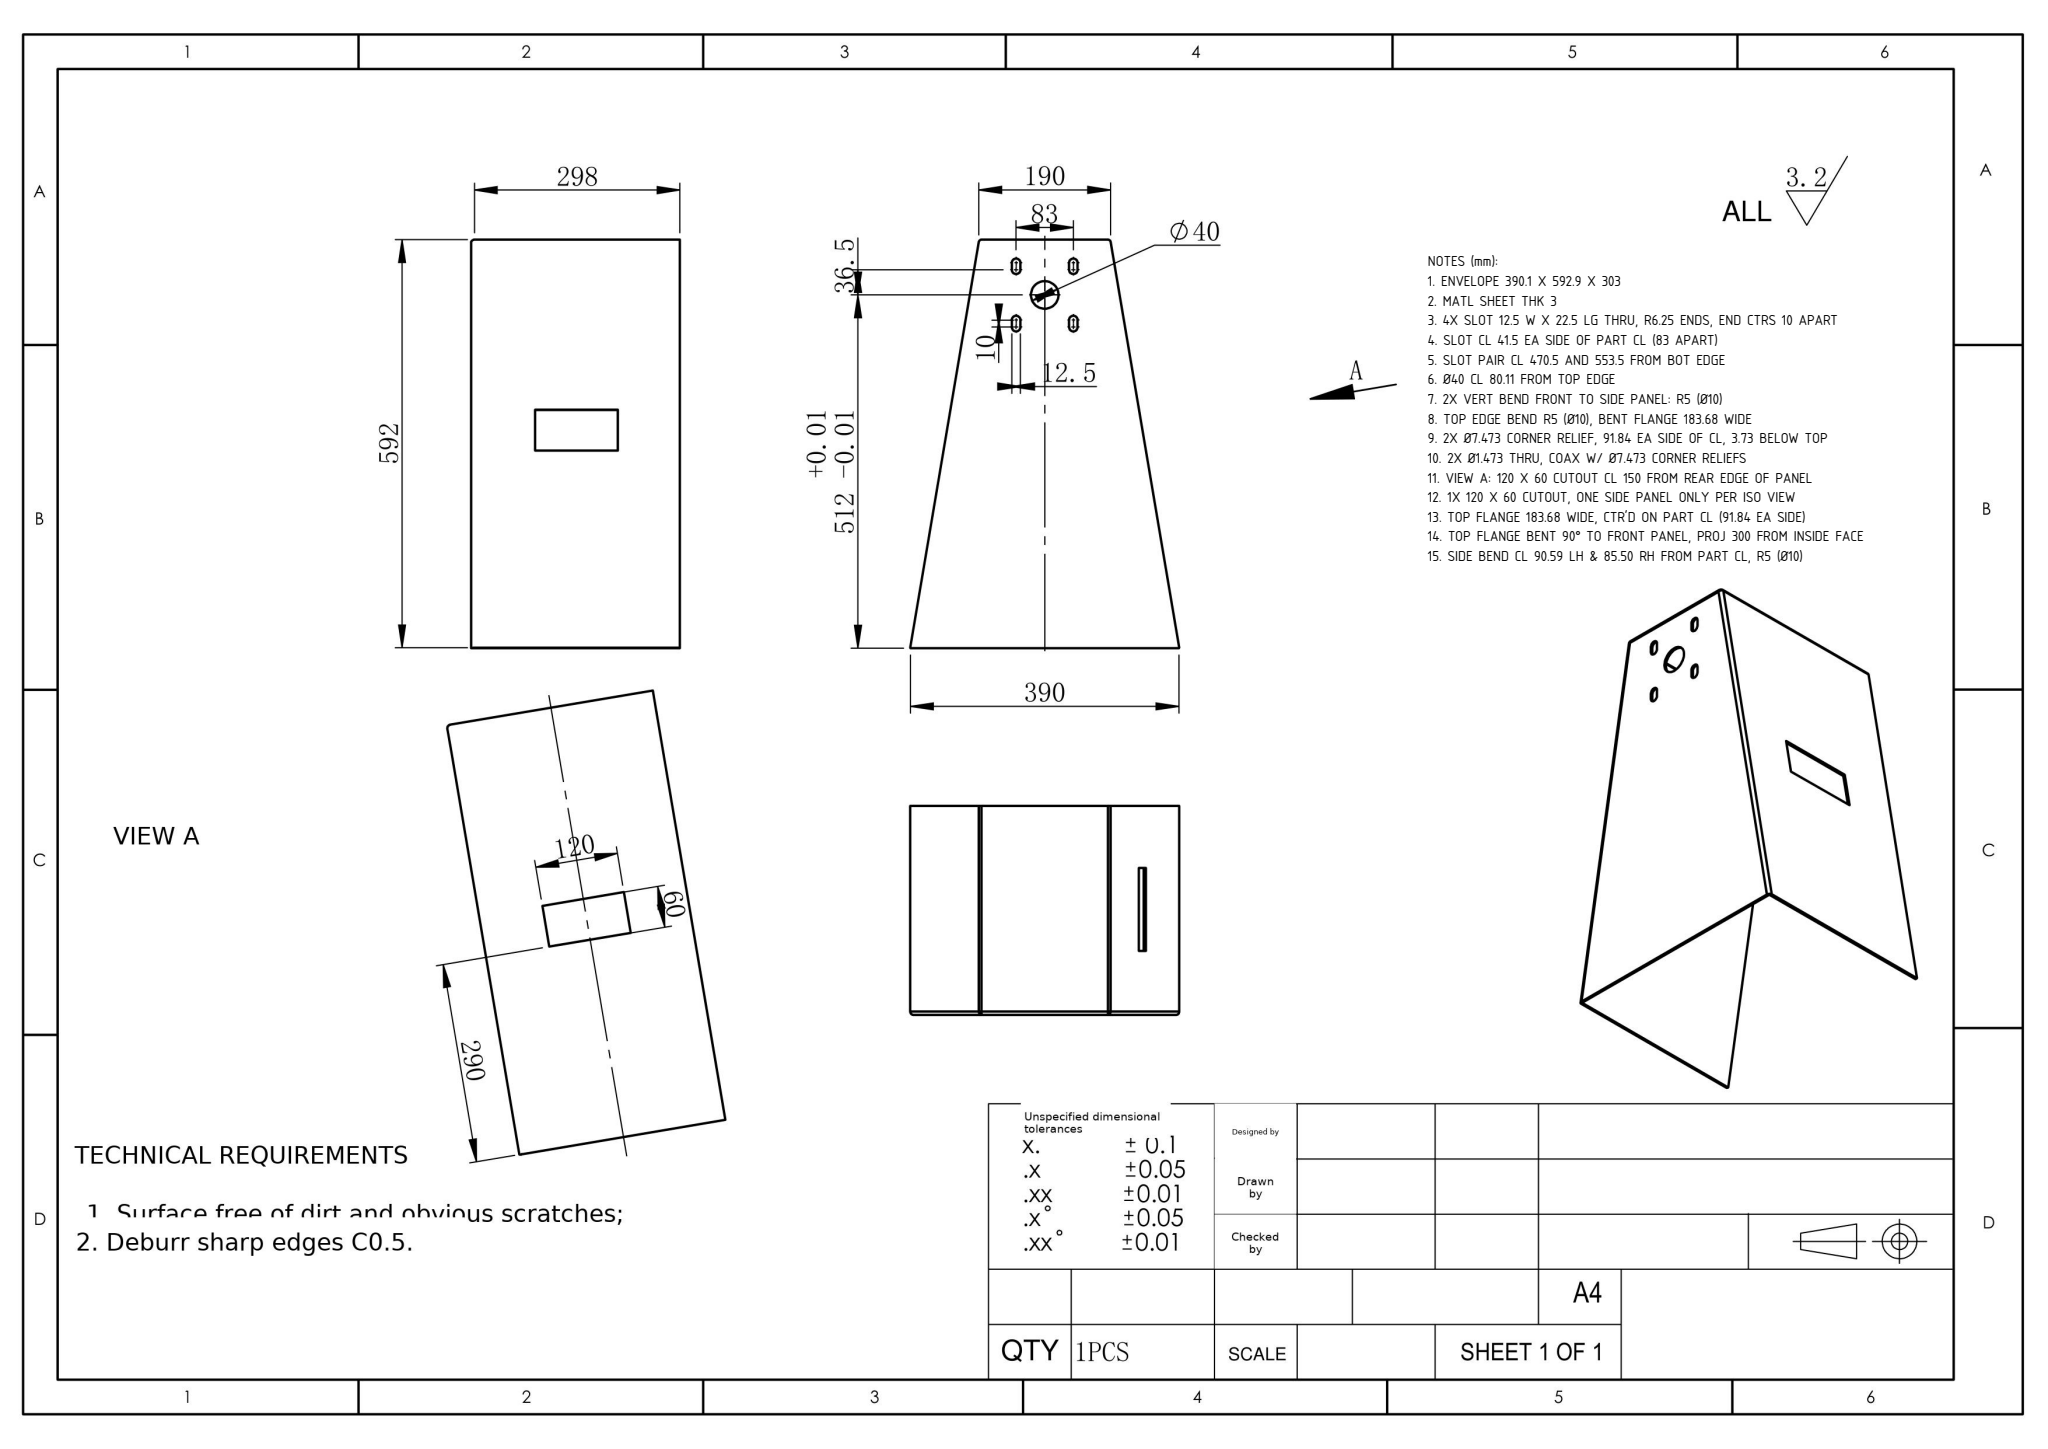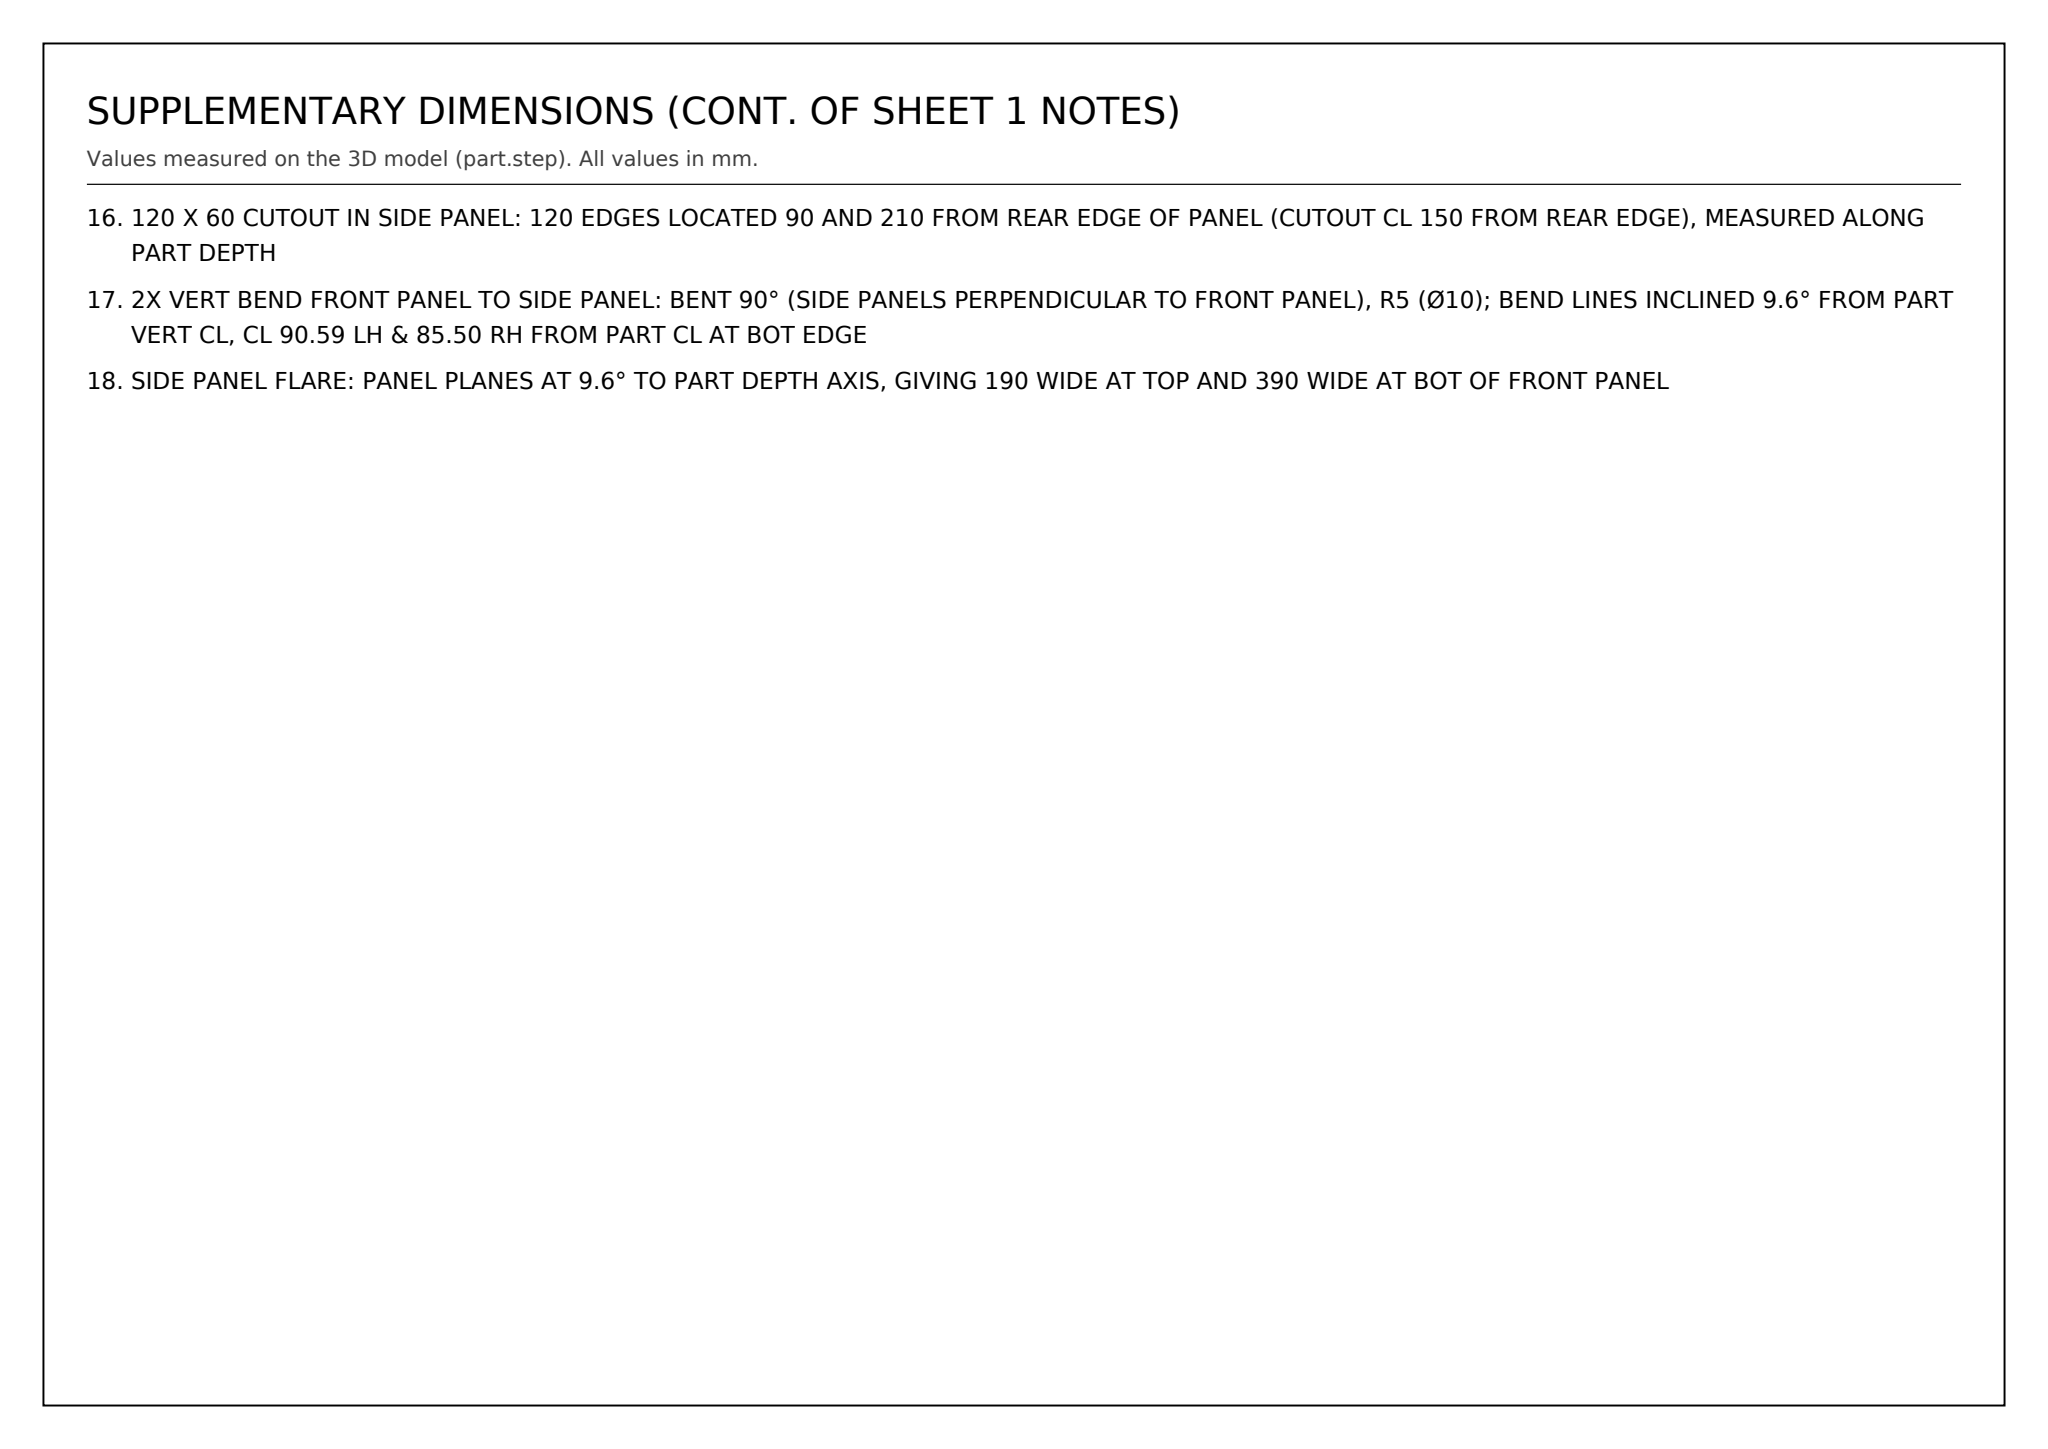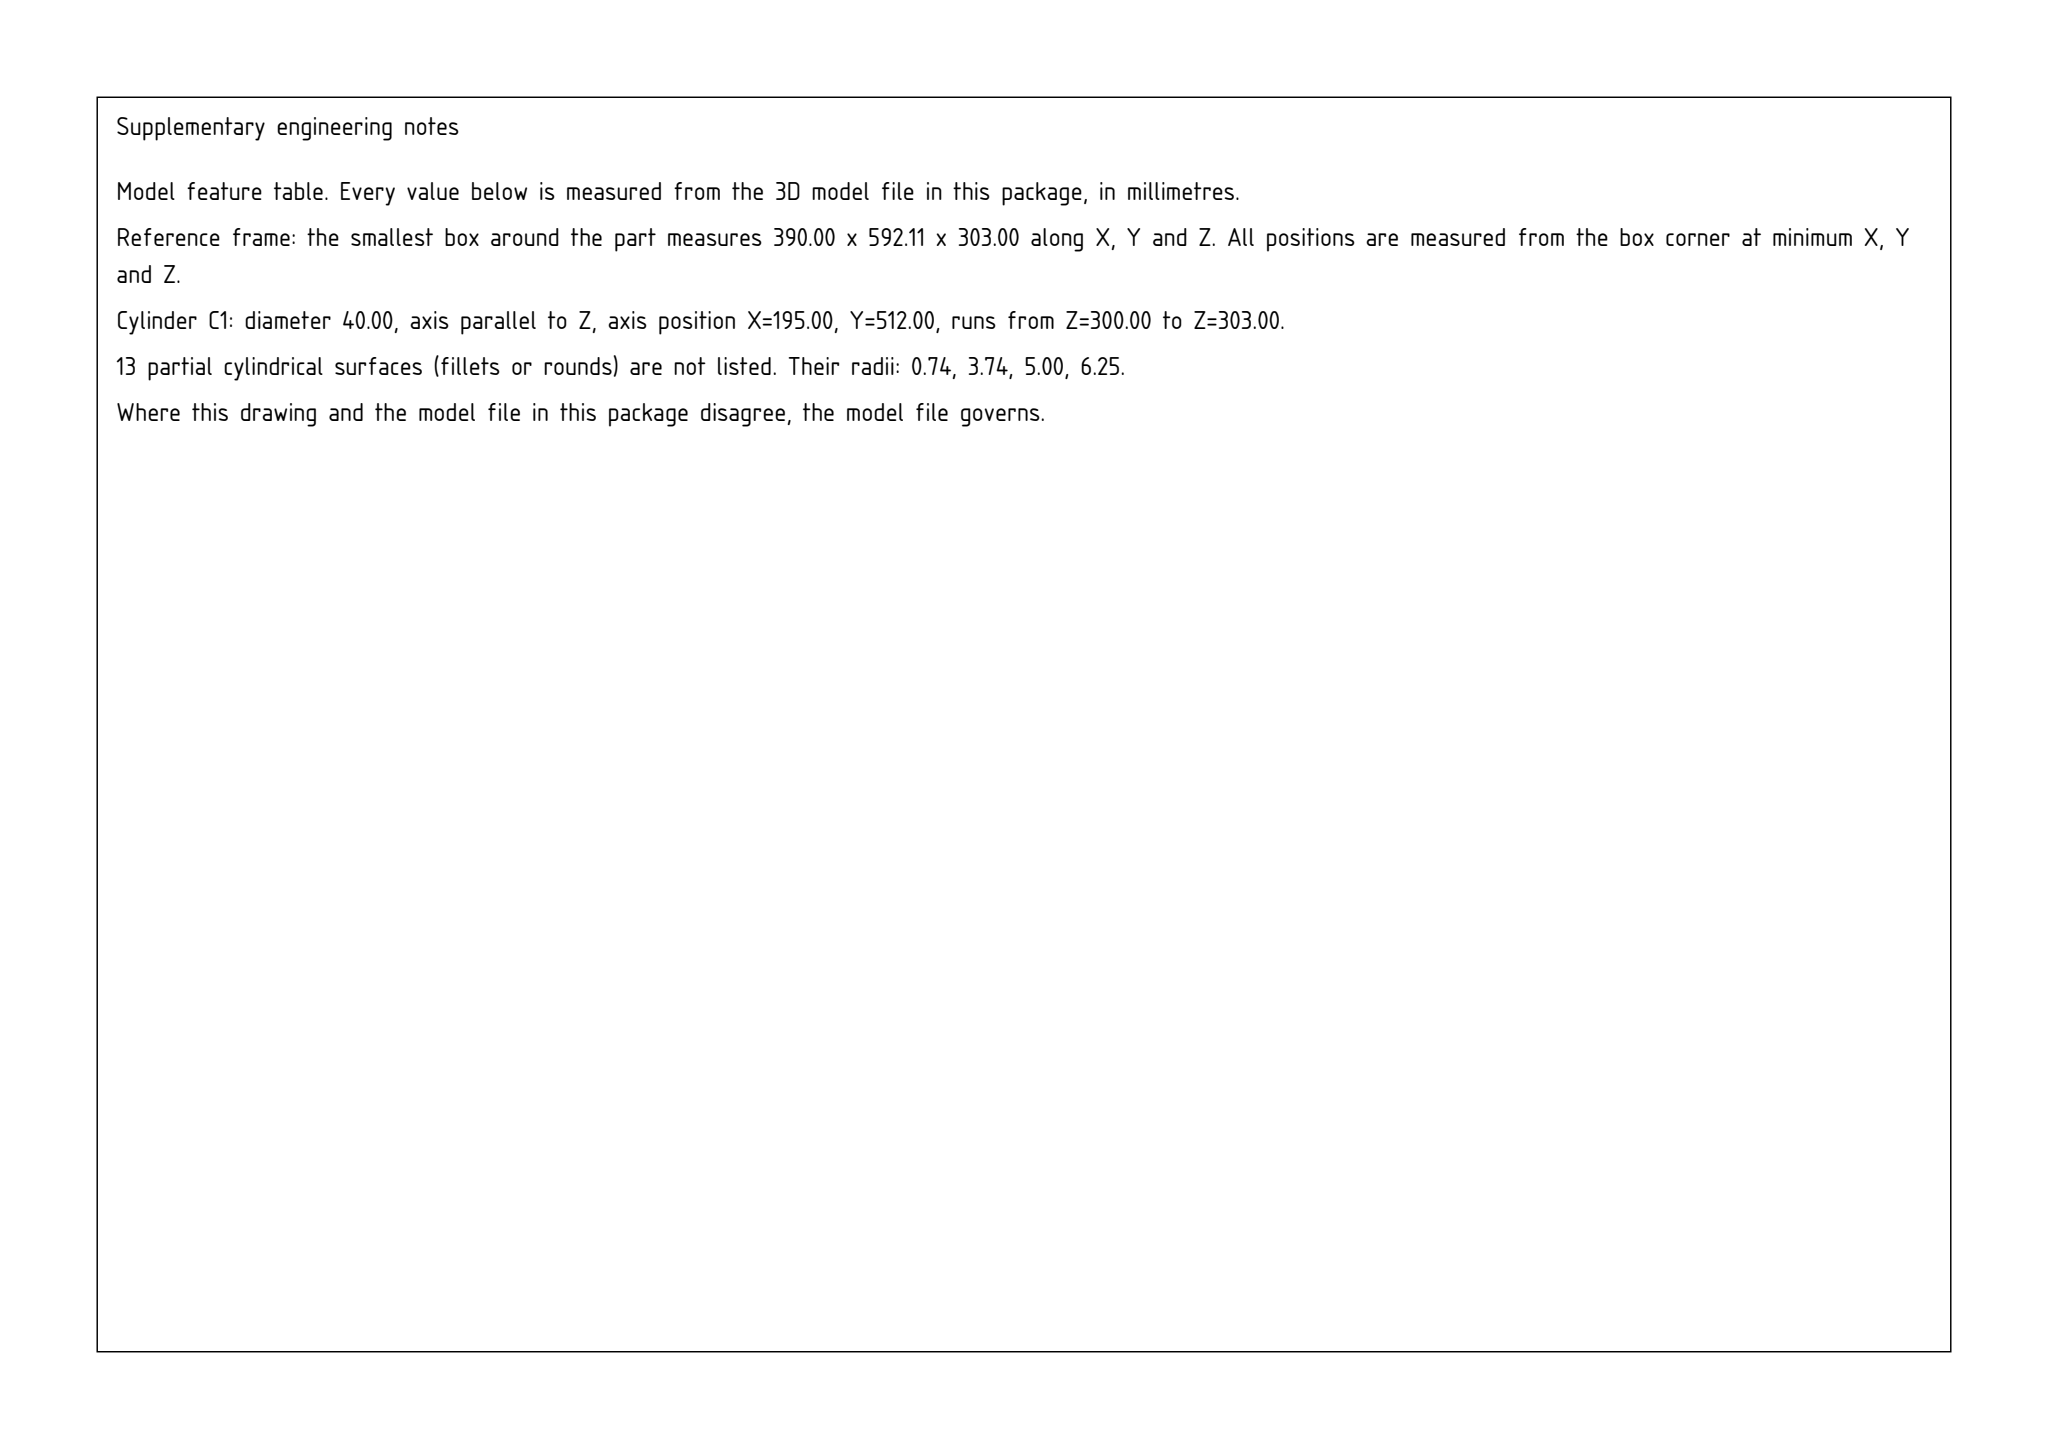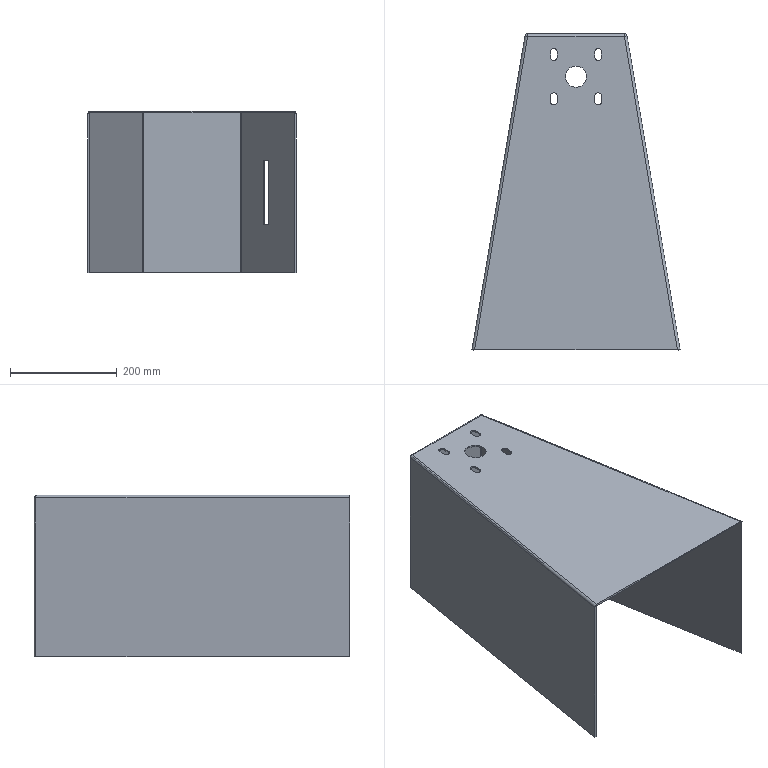Part | SolidWorks | mm | 1 solid | 49 faces | box 390 x 592.11 x 303 mm | volume 1724777 mm3 | plane 30 | cylinder 17 | spline 2 | commonest cylinder face diameters 12.5 x8 10 x3 40 x2 7.473 x2 1.473 x2
Drawing notes:
ENVELOPE 390.1 X 592.9 X 303 | from the solid: bbox_xyz 390.146 x 592.872 x 303.0
MATL SHEET THK 3 | from the solid: Z planes at 300 and 303 (3 apart); all hole cyls 3 long
4X SLOT 12.5 W X 22.5 LG THRU, R6.25 ENDS, END CTRS 10 APART | from the solid: 12.5 dia cyls paired at y 466.26/476.26 and 549.26/559.26; x planes 147.32/159.82 and 230.32/242.82 give 12.5 width; cyl length 3 = THK
SLOT CL 41.5 EA SIDE OF PART CL (83 APART) | from the solid: slot CLs x=153.57 & 236.57, part CL x=195.07 (Ø40 axis)
SLOT PAIR CL 470.5 AND 553.5 FROM BOT EDGE | from the solid: slot centers y=471.26 & 554.26; bottom edge plane y=0.76
Ø40 CL 80.11 FROM TOP EDGE | from the solid: 40 dia axis at y=512.76; top edge plane y=592.87
2X VERT BEND FRONT TO SIDE PANEL: R5 (Ø10) | from the solid: cylinders dia 10, axis y, at x=104.48 & x=280.57, z=298, len 589.76
TOP EDGE BEND R5 (Ø10), BENT FLANGE 183.68 WIDE | from the solid: cylinder dia 10, axis x, y=587.87, z=298, length 183.68; y planes 589.87/592.87
2X Ø7.473 CORNER RELIEF, 91.84 EA SIDE OF CL, 3.73 BELOW TOP | from the solid: Ø7.473 z-cyl at x=103.23 & 286.91, y=589.14; CL x=195.07 (Ø40), top y=592.87
2X Ø1.473 THRU, COAX W/ Ø7.473 CORNER RELIEFS | from the solid: Ø1.473 z-cyl at x=103.23 & 286.91, y=589.14, len 300
VIEW A: 120 X 60 CUTOUT CL 150 FROM REAR EDGE OF PANEL | from the solid: z planes at 90 and 210 (120 span, CL z=150); rear edge z=0
1X 120 X 60 CUTOUT, ONE SIDE PANEL ONLY PER ISO VIEW | from the solid: z=90 and z=210 planes each count 1 -> single cutout
TOP FLANGE 183.68 WIDE, CTR'D ON PART CL (91.84 EA SIDE) | from the solid: Ø10 bend cyl, axis x, y=587.87 z=298, length 183.68; flange side bend cyls at x=103.23 & 286.91, midpoint 195.07 = Ø40 hole CL (195.07)
TOP FLANGE BENT 90° TO FRONT PANEL, PROJ 300 FROM INSIDE FACE | from the solid: Flange faces are y-normal planes 589.87 & 592.87 (3 thk) vs front panel z-normal planes 300/303; flange edge bend cyls run z=300->0 (len 300) and z=298->0 (len 298); bbox z=303
SIDE BEND CL 90.59 LH & 85.50 RH FROM PART CL, R5 (Ø10) | from the solid: Ø10 cyls, axis y, len 589.76, at x=104.48 and x=280.57, z=298; part CL x=195.07 (Ø40 hole axis)
120 X 60 CUTOUT IN SIDE PANEL: 120 EDGES LOCATED 90 AND 210 FROM REAR EDGE OF PANEL (CUTOUT CL 150 FROM REAR EDGE), MEASURED ALONG PART DEPTH | from the solid: axis_planes normal z at offset 90 and 210 (120 apart, CL at 150 from z=0 rear face); bbox_xyz z = 303
2X VERT BEND FRONT PANEL TO SIDE PANEL: BENT 90° (SIDE PANELS PERPENDICULAR TO FRONT PANEL), R5 (Ø10); BEND LINES INCLINED 9.6° FROM PART VERT CL, CL 90.59 LH & 85.50 RH FROM PART CL AT BOT EDGE | from the solid: inclined_planes angle_to_xyz_axes [9.6, 80.4, 90.0] (side panel normals lie in XY plane, 90° to Z) vs front panel plane z=300 (normal Z); convex arc dia 10 'inclined' axis at x=104.5 and x=280.6, z=298
SIDE PANEL FLARE: PANEL PLANES AT 9.6° TO PART DEPTH AXIS, GIVING 190 WIDE AT TOP AND 390 WIDE AT BOT OF FRONT PANEL | from the solid: inclined_planes angle_to_xyz_axes [9.6, 80.4, 90.0], size [99.5, 588.5, 300.0]; bbox_xyz 390.146 x 592.872 x 303.0